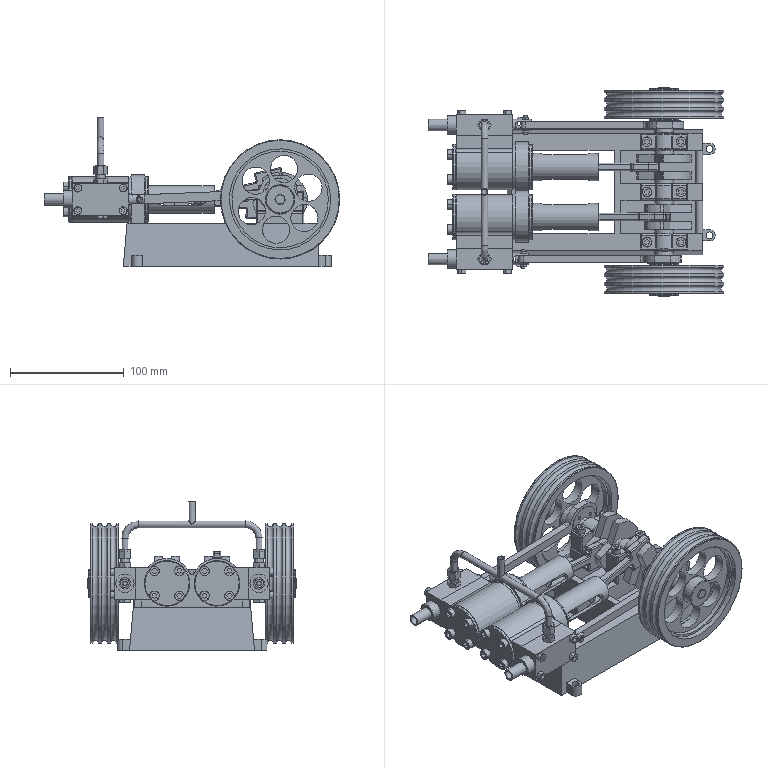Assembly | NX | mm | 82 component files | 82 solids | 1656 faces | box 260 x 184 x 131 mm | volume 789706 mm3 | plane 662 | cylinder 594 | cone 176 | torus 168 | sphere 52 | other 4 | commonest cylinder face diameters 2 x120 5 x90 4 x63 6 x38 10 x34 8.5 x28 3 x20 9 x19
Bill of materials:
unnamed part 1 | 2 |  | Hexagonal prism section joined coaxially to a plain cylindrical shank, with a through bore along the axis; hex outer end chamfered.
unnamed part 2 | 2 |  | Prismatic cylindrical body with a large central through bore, four smaller axial holes on a circle around it, and a rectangular block running the full length off one side, blended into the cylinder with fillets.
unnamed part 3 | 2 |  | Thin circular disc with four through holes near the rim and a shallow raised circular boss in the middle of one face; no central hole.
unnamed part 4 | 2 |  | Solid hexagonal base with chamfered edges on one face and a solid cylindrical boss standing coaxially on the other face.
unnamed part 5 | 2 |  | Hollow cylindrical tube with an integral hexagonal collar partway along its length; through bore along the full length.
unnamed part 6 | 2 |  | Stepped cylindrical shaft with two filleted reduced-diameter necks (one long, one short) and a forked end: an axial slot splits the end into two tines with a transverse hole through both.
unnamed part 7 | 2 |  | Solid stepped pin: a long central cylinder with a smaller-diameter cylindrical journal at each end; the two ends differ slightly in length and diameter.
unnamed part 8 | 4 |  | Thin flat annular ring with a rectangular cross-section and a relatively large inner diameter.
unnamed part 9 | 2 |  | Short cylindrical disc with a small central through bore and two rectangular circumferential grooves, leaving three raised lands.
unnamed part 10 | 14 |  | Cylindrical-head fastener-like shape: a cylindrical head with a hexagonal socket recess, a plain cylindrical shank narrower than the head, and a chamfered tip.
unnamed part 11 | 4 |  | Hexagonal prism with a central circular through hole and chamfered corners on both faces, giving curved chamfer arcs on each flat.
unnamed part 12 | 2 |  | Plain solid right circular cylinder with flat ends.
unnamed part 13 | 2 |  | Grooved wheel shaped like a pulley. It has three round-profile grooves around the rim, a flat web with six round lightening holes, and a central hub with a bore.
unnamed part 14 | 2 |  | Thin flat round disc with one large off-centre hole and two smaller holes.
unnamed part 15 | 2 |  | Long straight arm with a rounded eye and through-hole at one end. The other end is a thicker rectangular block with a semicircular cut-out on its end face and two through-holes on either side of it, shaped like half of a clamp.
unnamed part 16 | 2 |  | Thin flat lever plate, shaped like a spanner. A long straight handle has a small hole at its tip, and the other end is a ring with a large circular opening. The ring's outer edge is faceted with flats.
unnamed part 17 | 2 |  | Hexagonal prism shaped like a nut, with a plain central round bore and a chamfered top end that produces curved edges on the flats.
unnamed part 18 | 1 |  | Round tube bent into a U shape. It has a long straight crossbar, two radiused bends into parallel legs, and a short straight tube stub joined at the middle of the crossbar, pointing away from the legs.
unnamed part 19 | 2 |  | Solid stepped cylindrical shaft with a longer, larger-diameter centre section and a smaller-diameter journal of similar size at each end.
unnamed part 20 | 2 |  | Flanged hub or bushing. A round flange with four holes on a pitch circle carries a cylindrical boss with a central bore on one side and a short, shallow step on the other side.
unnamed part 21 | 2 |  | Plain straight cylindrical tube with constant wall thickness and square-cut ends.
unnamed part 22 | 2 |  | Clevis-like body: a round-based block with flats on two opposite sides and a curved top. Two parallel flat lugs with rounded ends and cross holes extend from one face, leaving a slot between them.
unnamed part 23 | 2 |  | Rectangular block with rounded edges, a semicircular cut-out on one long face and two parallel through-holes on either side of it, shaped like a clamp cap or half bearing block.
unnamed part 24 | 2 |  | Sharp-edged rectangular block with a cylindrical boss on one end. It has four corner holes through one large face, one cross hole through an adjacent face, and a large round bore in the end face opposite the boss.
unnamed part 25 | 2 |  | Circular flange disc with a cylindrical step on each face. On one face a smaller boss sits off-center and carries a through bore. On the other face the step is larger, close to the full disc diameter. The disc has two small through holes.
unnamed part 26 | 2 |  | Thin-walled cylindrical tube with a round flange at one end. The flange has four through holes evenly spaced around it. The tube wall has elongated, round-ended slots; at least one opposed pair passes right through.
unnamed part 27 | 3 |  | Rectangular block with filleted edges. A semicircular hump is raised in the middle of the top face. A horizontal through bore runs under the hump, and two vertical through holes sit near the block ends.
unnamed part 28 | 1 |  | Rectangular open frame or chassis with a large rectangular window. At one end, two upright lobed plates each carry a large central hole and a ring of smaller holes. The base has raised pads with paired holes, rod-like cylindrical features along one edge, and small mounting lugs with holes.
unnamed part 29 | 8 |  | Cylindrical-head screw-like part. It has a hexagonal socket recess in the head and a plain cylindrical shank with a chamfered tip.
unnamed part 30 | 2 |  | Plain annular ring (thick washer or spacer shape) with a concentric through bore and flat parallel faces.
unnamed part 31 | 1 |  | Crankshaft-like shaft. A straight cylindrical shaft carries two pairs of webs; each pair is joined by an offset pin, and the two pins sit on opposite sides of the axis. The webs have a partial-disc outline with a wedge-shaped cutaway.
Mates:
1. fix | base 1 component
2. concentric | bracket 3 edge | base 1 edge
3. parallel | bracket 3 face | base 1 face
4. concentric | base 1 edge | bracket 2 edge
5. parallel | bracket 2 face | base 1 face
6. concentric | bracket 1 edge | base 1 edge
7. parallel | bracket 1 face | base 1 face
8. concentric | lower_end_cap 2 edge | base 1 edge
9. concentric | lower_end_cap 2 edge | base 1 edge
10. concentric | external_piston_cylinder 2 edge | lower_end_cap 2 edge
11. parallel | external_piston_cylinder 2 face | base 1 face
12. concentric | base 1 edge | lower_end_cap 1 edge
13. concentric | lower_end_cap 1 edge | base 1 edge
14. concentric | external_piston_cylinder 1 edge | lower_end_cap 1 edge
15. parallel | external_piston_cylinder 1 face | base 1 face
16. concentric | upper_end_cap 2 edge | external_piston_cylinder 2 edge
17. concentric | upper_end_cap 2 edge | external_piston_cylinder 2 edge
18. concentric | external_piston_cylinder 1 edge | upper_end_cap 1 edge
19. concentric | upper_end_cap 1 edge | external_piston_cylinder 1 edge
20. concentric | side_piston_cylinder 2 arc | external_piston_cylinder 1 edge
21. parallel | side_piston_cylinder 2 face | external_piston_cylinder 1 face
22. concentric | side_piston_cylinder 1 arc | external_piston_cylinder 2 edge
23. parallel | side_piston_cylinder 1 face | external_piston_cylinder 2 face
24. touch align | vent_pipe 2 face | side_piston_cylinder 2 face
25. distance | vent_pipe 2 face | side_piston_cylinder 2 face
26. touch align | vent_pipe 1 face | side_piston_cylinder 1 face
27. distance | vent_pipe 1 face | side_piston_cylinder 1 face
28. concentric | washer 2 arc | lower_end_cap 1 edge
29. concentric | pipe_cap 2 edge | washer 2 edge
30. parallel | pipe_cap 2 face | base 1 face
31. concentric | washer 1 arc | lower_end_cap 2 edge
32. concentric | pipe_cap 1 edge | washer 1 edge
33. parallel | pipe_cap 1 face | base 1 face
34. concentric | connecting_rod_support 2 arc | base 1 edge
35. parallel | connecting_rod_support 2 face | base 1 face
36. concentric | connecting_rod_support 1 arc | base 1 edge
37. parallel | connecting_rod_support 1 face | base 1 face
38. touch align | crankshaft 1 face | bracket 2 face
39. center | crankshaft 1 face | crankshaft 1 face | connecting_rod_support 2 face
40. touch align | pulley 2 face | crankshaft 1 face
41. touch align | pulley 1 face | crankshaft 1 face
42. concentric | eccentric_side_plate 2 arc | eccentric 2 edge
43. touch align | eccentric_side_plate 2 face | eccentric 2 face
44. center | eccentric_side_plate 2 face | eccentric 2 face | side_piston_cylinder 1 face
45. distance | crankshaft 1 face | pulley 1 face
46. touch align | eccentric 2 face | crankshaft 1 face
47. concentric | eccentric_side_plate 1 edge | eccentric 1 edge
48. touch align | eccentric 1 face | eccentric_side_plate 1 face
49. touch align | eccentric_side_plate 1 face | crankshaft 1 face
50. center | eccentric 1 face | eccentric_side_plate 1 face | side_piston_cylinder 2 face
51. distance | crankshaft 1 face | pulley 2 face
52. concentric | piston_rod 2 edge | piston 2 arc
53. concentric | piston_ring 4 arc | piston 2 edge
54. concentric | piston_ring 3 arc | piston 2 edge
55. concentric | connecting_block 2 edge | piston_rod 2 edge
56. concentric | connecting_pin 2 edge | connecting_block 2 arc
57. touch align | piston_rod 2 face | connecting_rod_support 2 face
58. parallel | connecting_block 2 face | base 1 face
59. concentric | piston_rod 1 edge | piston 1 edge
60. concentric | piston_ring 2 arc | piston 1 edge
61. concentric | piston_ring 1 arc | piston 1 edge
62. concentric | piston_rod 1 edge | connecting_block 1 edge
63. concentric | connecting_pin 1 edge | connecting_block 1 arc
64. touch align | piston_rod 1 face | connecting_rod_support 1 face
65. parallel | connecting_block 1 face | connecting_block 2 face
66. concentric | connecting_rod_1_lower_block 2 arc | connecting_rod_1 2 arc
67. parallel | connecting_rod_1_lower_block 2 face | connecting_rod_1 2 face
68. touch align | connecting_rod_1_lower_block 2 face | crankshaft 1 face
69. center | connecting_rod_1 2 face | connecting_rod_1 2 face | crankshaft 1 face | crankshaft 1 face
70. touch align | connecting_rod_1 2 face | connecting_pin 1 face
71. concentric | connecting_rod_1_lower_block 1 arc | connecting_rod_1 1 arc
72. parallel | connecting_rod_1_lower_block 1 face | connecting_rod_1 1 face
73. touch align | connecting_rod_1 1 face | crankshaft 1 face
74. center | connecting_rod_1_lower_block 1 face | connecting_rod_1_lower_block 1 face | crankshaft 1 face | crankshaft 1 face
75. touch align | connecting_rod_1 1 face | connecting_pin 2 face
76. touch align | connecting_pin_2 2 face | external_piston 2 face
77. center | connecting_pin_2 2 face | connecting_pin_2 2 face | external_piston 2 face | external_piston 2 face
78. touch align | external_piston 2 face | side_piston_cylinder 2 face
79. touch align | connecting_pin_2 1 face | external_piston 1 face
80. center | connecting_pin_2 1 face | connecting_pin_2 1 face | external_piston 1 face | external_piston 1 face
81. touch align | external_piston 1 face | side_piston_cylinder 1 face
82. parallel | external_piston 1 face | side_piston_cylinder 1 face
83. parallel | external_piston 2 face | side_piston_cylinder 2 face
84. touch align | connecting_rod_2 2 face | eccentric 1 face
85. center | connecting_rod_2 2 face | connecting_rod_2 2 face | eccentric 1 face | eccentric_side_plate 1 face
86. touch align | connecting_rod_2 2 face | connecting_pin_2 2 face
87. touch align | connecting_rod_2 1 face | eccentric 2 face
88. center | connecting_rod_2 1 face | connecting_rod_2 1 face | eccentric 2 face | eccentric_side_plate 2 face
89. touch align | connecting_pin_2 1 face | connecting_rod_2 1 face
90. concentric | bolt 2 edge | side_piston_cylinder 2 edge
91. parallel | bolt 2 face | side_piston_cylinder 2 face
92. concentric | bolt 1 edge | side_piston_cylinder 1 edge
93. parallel | bolt 1 face | side_piston_cylinder 1 face
94. concentric | side_piston_cylinder 2 edge | pipe_cap_2 2 edge
95. parallel | pipe_cap_2 2 face | side_piston_cylinder 2 face
96. concentric | side_piston_cylinder 1 edge | pipe_cap_2 1 edge
97. parallel | pipe_cap_2 1 face | side_piston_cylinder 2 face
98. concentric | pipe_cap_2 1 edge | pipe_cap_3 2 edge
99. parallel | pipe_cap_3 2 face | pipe_cap_2 1 face
100. concentric | pipe_cap_2 2 edge | pipe_cap_3 1 edge
101. parallel | pipe_cap_3 1 face | pipe_cap_2 2 face
102. touch align | pipe 1 face | pipe_cap_3 2 face
103. touch align | pipe 1 face | pipe_cap_3 1 face
104. distance | pipe 1 face | external_piston_cylinder 1 face
105. concentric | hex_socket_screw_M5x25 14 edge | bracket 3 edge
106. concentric | hex_socket_screw_M5x25 13 edge | bracket 3 edge
107. concentric | hex_socket_screw_M5x25 12 edge | bracket 2 edge
108. concentric | hex_socket_screw_M5x25 11 | bracket 2 edge
109. concentric | hex_socket_screw_M5x25 10 edge | bracket 1 edge
110. concentric | hex_socket_screw_M5x25 9 edge | bracket 1 edge
111. concentric | hex_socket_screw_M5x25 8 edge | upper_end_cap 2 edge
112. concentric | hex_socket_screw_M5x25 7 edge | upper_end_cap 1 edge
113. bond | upper_end_cap 2 component | assembly component
114. bond | hex_socket_screw_M5x25 8 component | assembly component
115. bond | hex_socket_screw_M5x25 6 component | assembly component
116. bond | hex_socket_screw_M5x25 5 component | assembly component
117. bond | hex_socket_screw_M5x25 4 component | assembly component
118. circular | assembly datumaxis | assembly cartesiancoordinatesystem | assembly cartesiancoordinatesystem | assembly cartesiancoordinatesystem | assembly cartesiancoordinatesystem
119. bond | upper_end_cap 1 component | assembly component
120. bond | hex_socket_screw_M5x25 7 component | assembly component
121. bond | hex_socket_screw_M5x25 3 component | assembly component
122. bond | hex_socket_screw_M5x25 2 component | assembly component
123. bond | hex_socket_screw_M5x25 1 component | assembly component
124. circular | assembly datumaxis | assembly cartesiancoordinatesystem | assembly cartesiancoordinatesystem | assembly cartesiancoordinatesystem | assembly cartesiancoordinatesystem
125. concentric | hex_socket_screw_M4x25 8 edge | side_piston_cylinder 2 edge
126. concentric | hex_socket_screw_M4x25 7 edge | side_piston_cylinder 2 edge
127. concentric | hex_socket_screw_M4x25 6 edge | side_piston_cylinder 2 edge
128. concentric | hex_socket_screw_M4x25 5 edge | side_piston_cylinder 2 edge
129. concentric | hex_socket_screw_M4x25 4 edge | side_piston_cylinder 1 edge
130. concentric | hex_socket_screw_M4x25 3 edge | side_piston_cylinder 1 edge
131. concentric | hex_socket_screw_M4x25 2 edge | side_piston_cylinder 1 edge
132. concentric | hex_socket_screw_M4x25 1 edge | side_piston_cylinder 1 edge